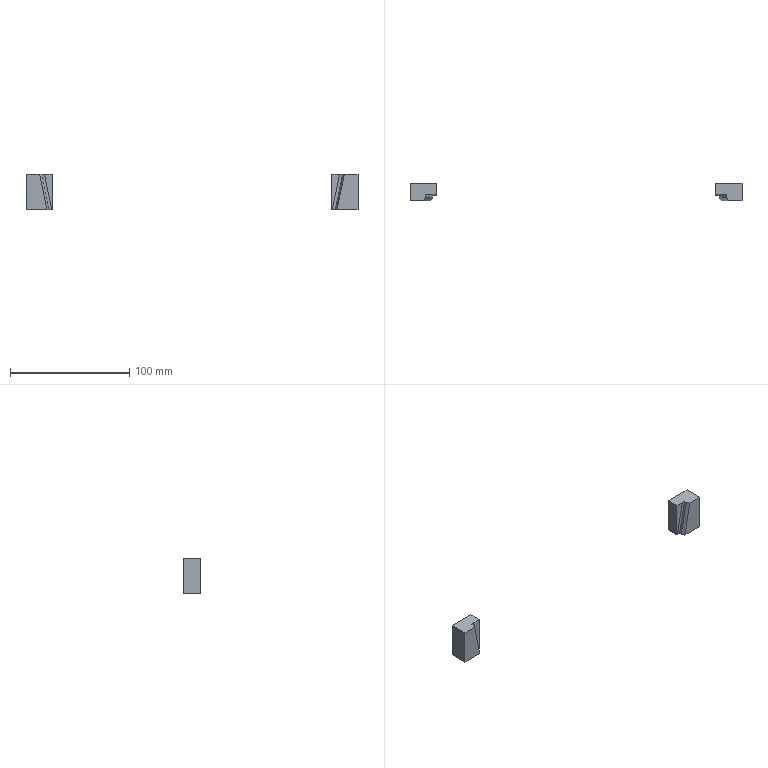Component | SolidWorks | Press-inFixture3-1 | 2 solids | 36 faces | box 278 x 15 x 30 mm | volume 17452 mm3 | plane 20 | cylinder 8 | cone 8 | commonest cylinder face diameters 3.3 x8
STEP:
#1=COLOUR_RGB('',0.7922,0.8196,0.9333);
#2=FILL_AREA_STYLE_COLOUR('',#1);
#3=FILL_AREA_STYLE('',(#2));
#4=SURFACE_STYLE_FILL_AREA(#3);
#5=SURFACE_SIDE_STYLE('',(#4));
#6=SURFACE_STYLE_USAGE(.BOTH.,#5);
#7=PRESENTATION_STYLE_ASSIGNMENT((#6));
#8=CARTESIAN_POINT('',(-3.99,-3.031,7.209));
#9=VERTEX_POINT('',#8);
#10=CARTESIAN_POINT('',(-4.12,-3.031,7.209));
#11=VERTEX_POINT('',#10);
#12=CARTESIAN_POINT('',(-4.055,-3.031,7.209));
#13=DIRECTION('',(-0.,1.,-0.));
#14=DIRECTION('',(-1.,0.,0.));
#15=AXIS2_PLACEMENT_3D('',#12,#13,#14);
#16=CIRCLE('',#15,0.06496);
#17=EDGE_CURVE('',#9,#11,#16,.T.);
#18=ORIENTED_EDGE('',*,*,#17,.F.);
#19=CARTESIAN_POINT('',(-3.99,-2.579,7.209));
#20=VERTEX_POINT('',#19);
#21=CARTESIAN_POINT('',(-3.99,-2.579,7.209));
#22=DIRECTION('',(-0.,1.,-0.));
#23=VECTOR('',#22,39.37);
#24=LINE('',#21,#23);
#25=EDGE_CURVE('',#9,#20,#24,.T.);
#26=ORIENTED_EDGE('',*,*,#25,.T.);
#27=CARTESIAN_POINT('',(-4.12,-2.579,7.209));
#28=VERTEX_POINT('',#27);
#29=CARTESIAN_POINT('',(-4.055,-2.579,7.209));
#30=DIRECTION('',(-0.,1.,-0.));
#31=DIRECTION('',(-1.,0.,0.));
#32=AXIS2_PLACEMENT_3D('',#29,#30,#31);
#33=CIRCLE('',#32,0.06496);
#34=EDGE_CURVE('',#20,#28,#33,.T.);
#35=ORIENTED_EDGE('',*,*,#34,.T.);
#36=CARTESIAN_POINT('',(-4.12,-2.579,7.209));
#37=DIRECTION('',(-0.,1.,-0.));
#38=VECTOR('',#37,39.37);
#39=LINE('',#36,#38);
#40=EDGE_CURVE('',#11,#28,#39,.T.);
#41=ORIENTED_EDGE('',*,*,#40,.F.);
#42=EDGE_LOOP('',(#18,#26,#35,#41));
#43=FACE_OUTER_BOUND('',#42,.T.);
#44=CARTESIAN_POINT('',(-4.055,-2.579,7.209));
#45=DIRECTION('',(-0.,1.,-0.));
#46=DIRECTION('',(-1.,0.,0.));
#47=AXIS2_PLACEMENT_3D('',#44,#45,#46);
#48=CYLINDRICAL_SURFACE('',#47,0.06496);
#49=ADVANCED_FACE('',(#43),#48,.F.);
#50=CARTESIAN_POINT('',(-4.055,-3.071,7.209));
#51=VERTEX_POINT('',#50);
#52=CARTESIAN_POINT('',(-4.12,-3.031,7.209));
#53=DIRECTION('',(-0.8572,0.515,0.));
#54=VECTOR('',#53,39.37);
#55=LINE('',#52,#54);
#56=EDGE_CURVE('',#51,#11,#55,.T.);
#57=ORIENTED_EDGE('',*,*,#56,.F.);
#58=CARTESIAN_POINT('',(-3.99,-3.031,7.209));
#59=DIRECTION('',(0.8572,0.515,-0.));
#60=VECTOR('',#59,39.37);
#61=LINE('',#58,#60);
#62=EDGE_CURVE('',#51,#9,#61,.T.);
#63=ORIENTED_EDGE('',*,*,#62,.T.);
#64=ORIENTED_EDGE('',*,*,#17,.T.);
#65=EDGE_LOOP('',(#57,#63,#64));
#66=FACE_OUTER_BOUND('',#65,.T.);
#67=CARTESIAN_POINT('',(-4.055,-3.031,7.209));
#68=DIRECTION('',(-0.,1.,-0.));
#69=DIRECTION('',(-1.,0.,0.));
#70=AXIS2_PLACEMENT_3D('',#67,#68,#69);
#71=CONICAL_SURFACE('',#70,0.06496,1.03);
#72=ADVANCED_FACE('',(#66),#71,.F.);
#73=CARTESIAN_POINT('',(-3.99,-3.031,6.658));
#74=VERTEX_POINT('',#73);
#75=CARTESIAN_POINT('',(-4.12,-3.031,6.658));
#76=VERTEX_POINT('',#75);
#77=CARTESIAN_POINT('',(-4.055,-3.031,6.658));
#78=DIRECTION('',(-0.,1.,-0.));
#79=DIRECTION('',(-1.,0.,0.));
#80=AXIS2_PLACEMENT_3D('',#77,#78,#79);
#81=CIRCLE('',#80,0.06496);
#82=EDGE_CURVE('',#74,#76,#81,.T.);
#83=ORIENTED_EDGE('',*,*,#82,.F.);
#84=CARTESIAN_POINT('',(-3.99,-2.579,6.658));
#85=VERTEX_POINT('',#84);
#86=CARTESIAN_POINT('',(-3.99,-2.579,6.658));
#87=DIRECTION('',(-0.,1.,-0.));
#88=VECTOR('',#87,39.37);
#89=LINE('',#86,#88);
#90=EDGE_CURVE('',#74,#85,#89,.T.);
#91=ORIENTED_EDGE('',*,*,#90,.T.);
#92=CARTESIAN_POINT('',(-4.12,-2.579,6.658));
#93=VERTEX_POINT('',#92);
#94=CARTESIAN_POINT('',(-4.055,-2.579,6.658));
#95=DIRECTION('',(-0.,1.,-0.));
#96=DIRECTION('',(-1.,0.,0.));
#97=AXIS2_PLACEMENT_3D('',#94,#95,#96);
#98=CIRCLE('',#97,0.06496);
#99=EDGE_CURVE('',#85,#93,#98,.T.);
#100=ORIENTED_EDGE('',*,*,#99,.T.);
#101=CARTESIAN_POINT('',(-4.12,-2.579,6.658));
#102=DIRECTION('',(-0.,1.,-0.));
#103=VECTOR('',#102,39.37);
#104=LINE('',#101,#103);
#105=EDGE_CURVE('',#76,#93,#104,.T.);
#106=ORIENTED_EDGE('',*,*,#105,.F.);
#107=EDGE_LOOP('',(#83,#91,#100,#106));
#108=FACE_OUTER_BOUND('',#107,.T.);
#109=CARTESIAN_POINT('',(-4.055,-2.579,6.658));
#110=DIRECTION('',(-0.,1.,-0.));
#111=DIRECTION('',(-1.,0.,0.));
#112=AXIS2_PLACEMENT_3D('',#109,#110,#111);
#113=CYLINDRICAL_SURFACE('',#112,0.06496);
#114=ADVANCED_FACE('',(#108),#113,.F.);
#115=CARTESIAN_POINT('',(-4.055,-3.071,6.658));
#116=VERTEX_POINT('',#115);
#117=CARTESIAN_POINT('',(-4.12,-3.031,6.658));
#118=DIRECTION('',(-0.8572,0.515,0.));
#119=VECTOR('',#118,39.37);
#120=LINE('',#117,#119);
#121=EDGE_CURVE('',#116,#76,#120,.T.);
#122=ORIENTED_EDGE('',*,*,#121,.F.);
#123=CARTESIAN_POINT('',(-3.99,-3.031,6.658));
#124=DIRECTION('',(0.8572,0.515,-0.));
#125=VECTOR('',#124,39.37);
#126=LINE('',#123,#125);
#127=EDGE_CURVE('',#116,#74,#126,.T.);
#128=ORIENTED_EDGE('',*,*,#127,.T.);
#129=ORIENTED_EDGE('',*,*,#82,.T.);
#130=EDGE_LOOP('',(#122,#128,#129));
#131=FACE_OUTER_BOUND('',#130,.T.);
#132=CARTESIAN_POINT('',(-4.055,-3.031,6.658));
#133=DIRECTION('',(-0.,1.,-0.));
#134=DIRECTION('',(-1.,0.,0.));
#135=AXIS2_PLACEMENT_3D('',#132,#133,#134);
#136=CONICAL_SURFACE('',#135,0.06496,1.03);
#137=ADVANCED_FACE('',(#131),#136,.F.);
#138=CARTESIAN_POINT('',(-3.545,-2.972,6.343));
#139=VERTEX_POINT('',#138);
#140=CARTESIAN_POINT('',(-3.544,-3.051,6.343));
#141=VERTEX_POINT('',#140);
#142=CARTESIAN_POINT('',(-3.542,-3.171,6.343));
#143=DIRECTION('',(0.01741,-0.9998,0.));
#144=VECTOR('',#143,39.37);
#145=LINE('',#142,#144);
#146=EDGE_CURVE('',#139,#141,#145,.T.);
#147=ORIENTED_EDGE('',*,*,#146,.T.);
#148=CARTESIAN_POINT('',(-3.602,-3.169,6.343));
#149=VERTEX_POINT('',#148);
#150=CARTESIAN_POINT('',(-3.6,-3.164,6.343));
#151=DIRECTION('',(-0.4419,-0.8971,0.));
#152=VECTOR('',#151,39.37);
#153=LINE('',#150,#152);
#154=EDGE_CURVE('',#141,#149,#153,.T.);
#155=ORIENTED_EDGE('',*,*,#154,.T.);
#156=CARTESIAN_POINT('',(-4.291,-3.169,6.343));
#157=VERTEX_POINT('',#156);
#158=CARTESIAN_POINT('',(-3.425,-3.169,6.343));
#159=DIRECTION('',(1.,0.,-0.));
#160=VECTOR('',#159,39.37);
#161=LINE('',#158,#160);
#162=EDGE_CURVE('',#157,#149,#161,.T.);
#163=ORIENTED_EDGE('',*,*,#162,.F.);
#164=CARTESIAN_POINT('',(-4.291,-2.579,6.343));
#165=VERTEX_POINT('',#164);
#166=CARTESIAN_POINT('',(-4.291,-3.169,6.343));
#167=DIRECTION('',(-0.,1.,-0.));
#168=VECTOR('',#167,39.37);
#169=LINE('',#166,#168);
#170=EDGE_CURVE('',#157,#165,#169,.T.);
#171=ORIENTED_EDGE('',*,*,#170,.T.);
#172=CARTESIAN_POINT('',(-3.425,-2.579,6.343));
#173=VERTEX_POINT('',#172);
#174=CARTESIAN_POINT('',(-3.425,-2.579,6.343));
#175=DIRECTION('',(1.,0.,-0.));
#176=VECTOR('',#175,39.37);
#177=LINE('',#174,#176);
#178=EDGE_CURVE('',#165,#173,#177,.T.);
#179=ORIENTED_EDGE('',*,*,#178,.T.);
#180=CARTESIAN_POINT('',(-3.425,-2.972,6.343));
#181=VERTEX_POINT('',#180);
#182=CARTESIAN_POINT('',(-3.425,-3.169,6.343));
#183=DIRECTION('',(-0.,1.,-0.));
#184=VECTOR('',#183,39.37);
#185=LINE('',#182,#184);
#186=EDGE_CURVE('',#181,#173,#185,.T.);
#187=ORIENTED_EDGE('',*,*,#186,.F.);
#188=CARTESIAN_POINT('',(-3.445,-2.972,6.343));
#189=VERTEX_POINT('',#188);
#190=CARTESIAN_POINT('',(-3.425,-2.972,6.343));
#191=DIRECTION('',(-1.,0.,0.));
#192=VECTOR('',#191,39.37);
#193=LINE('',#190,#192);
#194=EDGE_CURVE('',#181,#189,#193,.T.);
#195=ORIENTED_EDGE('',*,*,#194,.T.);
#196=CARTESIAN_POINT('',(-3.425,-2.972,6.343));
#197=DIRECTION('',(1.,-0.,-0.));
#198=VECTOR('',#197,39.37);
#199=LINE('',#196,#198);
#200=EDGE_CURVE('',#139,#189,#199,.T.);
#201=ORIENTED_EDGE('',*,*,#200,.F.);
#202=EDGE_LOOP('',(#147,#155,#163,#171,#179,#187,#195,#201));
#203=FACE_OUTER_BOUND('',#202,.T.);
#204=CARTESIAN_POINT('',(-3.425,-3.169,6.343));
#205=DIRECTION('',(0.,0.,1.));
#206=DIRECTION('',(-1.,-0.,0.));
#207=AXIS2_PLACEMENT_3D('',#204,#205,#206);
#208=PLANE('',#207);
#209=ADVANCED_FACE('',(#203),#208,.F.);
#210=CARTESIAN_POINT('',(-3.425,-2.972,7.524));
#211=VERTEX_POINT('',#210);
#212=CARTESIAN_POINT('',(-3.425,-2.579,7.524));
#213=VERTEX_POINT('',#212);
#214=CARTESIAN_POINT('',(-3.425,-3.169,7.524));
#215=DIRECTION('',(-0.,1.,-0.));
#216=VECTOR('',#215,39.37);
#217=LINE('',#214,#216);
#218=EDGE_CURVE('',#211,#213,#217,.T.);
#219=ORIENTED_EDGE('',*,*,#218,.F.);
#220=CARTESIAN_POINT('',(-3.425,-2.972,7.524));
#221=DIRECTION('',(0.,0.,-1.));
#222=VECTOR('',#221,39.37);
#223=LINE('',#220,#222);
#224=EDGE_CURVE('',#211,#181,#223,.T.);
#225=ORIENTED_EDGE('',*,*,#224,.T.);
#226=ORIENTED_EDGE('',*,*,#186,.T.);
#227=CARTESIAN_POINT('',(-3.425,-2.579,7.524));
#228=DIRECTION('',(-0.,0.,1.));
#229=VECTOR('',#228,39.37);
#230=LINE('',#227,#229);
#231=EDGE_CURVE('',#173,#213,#230,.T.);
#232=ORIENTED_EDGE('',*,*,#231,.T.);
#233=EDGE_LOOP('',(#219,#225,#226,#232));
#234=FACE_OUTER_BOUND('',#233,.T.);
#235=CARTESIAN_POINT('',(-3.425,-3.169,7.524));
#236=DIRECTION('',(-1.,-0.,-0.));
#237=DIRECTION('',(0.,-0.,-1.));
#238=AXIS2_PLACEMENT_3D('',#235,#236,#237);
#239=PLANE('',#238);
#240=ADVANCED_FACE('',(#234),#239,.F.);
#241=CARTESIAN_POINT('',(-3.839,-3.169,7.524));
#242=VERTEX_POINT('',#241);
#243=CARTESIAN_POINT('',(-4.291,-3.169,7.524));
#244=VERTEX_POINT('',#243);
#245=CARTESIAN_POINT('',(-3.425,-3.169,7.524));
#246=DIRECTION('',(-1.,-0.,0.));
#247=VECTOR('',#246,39.37);
#248=LINE('',#245,#247);
#249=EDGE_CURVE('',#242,#244,#248,.T.);
#250=ORIENTED_EDGE('',*,*,#249,.F.);
#251=CARTESIAN_POINT('',(-3.781,-3.051,7.524));
#252=VERTEX_POINT('',#251);
#253=CARTESIAN_POINT('',(-3.79,-3.07,7.524));
#254=DIRECTION('',(0.4419,0.8971,-0.));
#255=VECTOR('',#254,39.37);
#256=LINE('',#253,#255);
#257=EDGE_CURVE('',#242,#252,#256,.T.);
#258=ORIENTED_EDGE('',*,*,#257,.T.);
#259=CARTESIAN_POINT('',(-3.782,-2.972,7.524));
#260=VERTEX_POINT('',#259);
#261=CARTESIAN_POINT('',(-3.779,-3.175,7.524));
#262=DIRECTION('',(-0.01741,0.9998,-0.));
#263=VECTOR('',#262,39.37);
#264=LINE('',#261,#263);
#265=EDGE_CURVE('',#252,#260,#264,.T.);
#266=ORIENTED_EDGE('',*,*,#265,.T.);
#267=CARTESIAN_POINT('',(-3.682,-2.972,7.524));
#268=VERTEX_POINT('',#267);
#269=CARTESIAN_POINT('',(-3.425,-2.972,7.524));
#270=DIRECTION('',(-1.,0.,0.));
#271=VECTOR('',#270,39.37);
#272=LINE('',#269,#271);
#273=EDGE_CURVE('',#268,#260,#272,.T.);
#274=ORIENTED_EDGE('',*,*,#273,.F.);
#275=CARTESIAN_POINT('',(-3.425,-2.972,7.524));
#276=DIRECTION('',(1.,-0.,-0.));
#277=VECTOR('',#276,39.37);
#278=LINE('',#275,#277);
#279=EDGE_CURVE('',#268,#211,#278,.T.);
#280=ORIENTED_EDGE('',*,*,#279,.T.);
#281=ORIENTED_EDGE('',*,*,#218,.T.);
#282=CARTESIAN_POINT('',(-4.291,-2.579,7.524));
#283=VERTEX_POINT('',#282);
#284=CARTESIAN_POINT('',(-3.425,-2.579,7.524));
#285=DIRECTION('',(-1.,-0.,0.));
#286=VECTOR('',#285,39.37);
#287=LINE('',#284,#286);
#288=EDGE_CURVE('',#213,#283,#287,.T.);
#289=ORIENTED_EDGE('',*,*,#288,.T.);
#290=CARTESIAN_POINT('',(-4.291,-3.169,7.524));
#291=DIRECTION('',(-0.,1.,-0.));
#292=VECTOR('',#291,39.37);
#293=LINE('',#290,#292);
#294=EDGE_CURVE('',#244,#283,#293,.T.);
#295=ORIENTED_EDGE('',*,*,#294,.F.);
#296=EDGE_LOOP('',(#250,#258,#266,#274,#280,#281,#289,#295));
#297=FACE_OUTER_BOUND('',#296,.T.);
#298=CARTESIAN_POINT('',(-3.425,-3.169,7.524));
#299=DIRECTION('',(-0.,-0.,-1.));
#300=DIRECTION('',(1.,0.,-0.));
#301=AXIS2_PLACEMENT_3D('',#298,#299,#300);
#302=PLANE('',#301);
#303=ADVANCED_FACE('',(#297),#302,.F.);
#304=CARTESIAN_POINT('',(-4.291,-2.579,7.524));
#305=DIRECTION('',(0.,-0.,-1.));
#306=VECTOR('',#305,39.37);
#307=LINE('',#304,#306);
#308=EDGE_CURVE('',#283,#165,#307,.T.);
#309=ORIENTED_EDGE('',*,*,#308,.T.);
#310=ORIENTED_EDGE('',*,*,#170,.F.);
#311=CARTESIAN_POINT('',(-4.291,-3.169,7.524));
#312=DIRECTION('',(0.,-0.,-1.));
#313=VECTOR('',#312,39.37);
#314=LINE('',#311,#313);
#315=EDGE_CURVE('',#244,#157,#314,.T.);
#316=ORIENTED_EDGE('',*,*,#315,.F.);
#317=ORIENTED_EDGE('',*,*,#294,.T.);
#318=EDGE_LOOP('',(#309,#310,#316,#317));
#319=FACE_OUTER_BOUND('',#318,.T.);
#320=CARTESIAN_POINT('',(-4.291,-3.169,7.524));
#321=DIRECTION('',(1.,0.,0.));
#322=DIRECTION('',(-0.,0.,1.));
#323=AXIS2_PLACEMENT_3D('',#320,#321,#322);
#324=PLANE('',#323);
#325=ADVANCED_FACE('',(#319),#324,.F.);
#326=ORIENTED_EDGE('',*,*,#162,.T.);
#327=CARTESIAN_POINT('',(-3.837,-3.169,7.512));
#328=DIRECTION('',(-0.1967,0.,0.9805));
#329=VECTOR('',#328,39.37);
#330=LINE('',#327,#329);
#331=EDGE_CURVE('',#149,#242,#330,.T.);
#332=ORIENTED_EDGE('',*,*,#331,.T.);
#333=ORIENTED_EDGE('',*,*,#249,.T.);
#334=ORIENTED_EDGE('',*,*,#315,.T.);
#335=EDGE_LOOP('',(#326,#332,#333,#334));
#336=FACE_OUTER_BOUND('',#335,.T.);
#337=CARTESIAN_POINT('',(-3.858,-3.169,6.933));
#338=DIRECTION('',(0.,-1.,0.));
#339=DIRECTION('',(1.,0.,-0.));
#340=AXIS2_PLACEMENT_3D('',#337,#338,#339);
#341=PLANE('',#340);
#342=ADVANCED_FACE('',(#336),#341,.T.);
#343=CARTESIAN_POINT('',(-4.055,-2.579,7.209));
#344=DIRECTION('',(-0.,1.,-0.));
#345=DIRECTION('',(-1.,0.,0.));
#346=AXIS2_PLACEMENT_3D('',#343,#344,#345);
#347=CIRCLE('',#346,0.06496);
#348=EDGE_CURVE('',#28,#20,#347,.T.);
#349=ORIENTED_EDGE('',*,*,#348,.F.);
#350=ORIENTED_EDGE('',*,*,#34,.F.);
#351=EDGE_LOOP('',(#349,#350));
#352=FACE_BOUND('',#351,.T.);
#353=CARTESIAN_POINT('',(-4.055,-2.579,6.658));
#354=DIRECTION('',(-0.,1.,-0.));
#355=DIRECTION('',(-1.,0.,0.));
#356=AXIS2_PLACEMENT_3D('',#353,#354,#355);
#357=CIRCLE('',#356,0.06496);
#358=EDGE_CURVE('',#93,#85,#357,.T.);
#359=ORIENTED_EDGE('',*,*,#358,.F.);
#360=ORIENTED_EDGE('',*,*,#99,.F.);
#361=EDGE_LOOP('',(#359,#360));
#362=FACE_BOUND('',#361,.T.);
#363=ORIENTED_EDGE('',*,*,#178,.F.);
#364=ORIENTED_EDGE('',*,*,#308,.F.);
#365=ORIENTED_EDGE('',*,*,#288,.F.);
#366=ORIENTED_EDGE('',*,*,#231,.F.);
#367=EDGE_LOOP('',(#363,#364,#365,#366));
#368=FACE_OUTER_BOUND('',#367,.T.);
#369=CARTESIAN_POINT('',(-3.858,-2.579,6.933));
#370=DIRECTION('',(0.,-1.,0.));
#371=DIRECTION('',(1.,0.,-0.));
#372=AXIS2_PLACEMENT_3D('',#369,#370,#371);
#373=PLANE('',#372);
#374=ADVANCED_FACE('',(#352,#362,#368),#373,.F.);
#375=ORIENTED_EDGE('',*,*,#194,.F.);
#376=ORIENTED_EDGE('',*,*,#224,.F.);
#377=ORIENTED_EDGE('',*,*,#279,.F.);
#378=CARTESIAN_POINT('',(-3.747,-2.972,7.85));
#379=DIRECTION('',(-0.1967,0.,0.9805));
#380=VECTOR('',#379,39.37);
#381=LINE('',#378,#380);
#382=EDGE_CURVE('',#189,#268,#381,.T.);
#383=ORIENTED_EDGE('',*,*,#382,.F.);
#384=EDGE_LOOP('',(#375,#376,#377,#383));
#385=FACE_OUTER_BOUND('',#384,.T.);
#386=CARTESIAN_POINT('',(-3.355,-2.972,6.018));
#387=DIRECTION('',(0.,1.,0.));
#388=DIRECTION('',(1.,-0.,0.));
#389=AXIS2_PLACEMENT_3D('',#386,#387,#388);
#390=PLANE('',#389);
#391=ADVANCED_FACE('',(#385),#390,.F.);
#392=CARTESIAN_POINT('',(-3.83,-2.972,7.763));
#393=DIRECTION('',(0.1967,-0.,-0.9805));
#394=VECTOR('',#393,39.37);
#395=LINE('',#392,#394);
#396=EDGE_CURVE('',#260,#139,#395,.T.);
#397=ORIENTED_EDGE('',*,*,#396,.T.);
#398=ORIENTED_EDGE('',*,*,#200,.T.);
#399=ORIENTED_EDGE('',*,*,#382,.T.);
#400=ORIENTED_EDGE('',*,*,#273,.T.);
#401=EDGE_LOOP('',(#397,#398,#399,#400));
#402=FACE_OUTER_BOUND('',#401,.T.);
#403=CARTESIAN_POINT('',(-1.579,-2.972,7.058));
#404=DIRECTION('',(-0.,-1.,0.));
#405=DIRECTION('',(-0.,0.,1.));
#406=AXIS2_PLACEMENT_3D('',#403,#404,#405);
#407=PLANE('',#406);
#408=ADVANCED_FACE('',(#402),#407,.T.);
#409=ORIENTED_EDGE('',*,*,#265,.F.);
#410=CARTESIAN_POINT('',(-3.544,-3.051,6.342));
#411=DIRECTION('',(0.1967,-0.,-0.9805));
#412=VECTOR('',#411,39.37);
#413=LINE('',#410,#412);
#414=EDGE_CURVE('',#252,#141,#413,.T.);
#415=ORIENTED_EDGE('',*,*,#414,.T.);
#416=ORIENTED_EDGE('',*,*,#146,.F.);
#417=ORIENTED_EDGE('',*,*,#396,.F.);
#418=EDGE_LOOP('',(#409,#415,#416,#417));
#419=FACE_OUTER_BOUND('',#418,.T.);
#420=CARTESIAN_POINT('',(-3.798,-4.876,7.765));
#421=DIRECTION('',(-0.9803,-0.01707,-0.1966));
#422=DIRECTION('',(-0.01745,0.9998,0.000201));
#423=AXIS2_PLACEMENT_3D('',#420,#421,#422);
#424=PLANE('',#423);
#425=ADVANCED_FACE('',(#419),#424,.F.);
#426=ORIENTED_EDGE('',*,*,#127,.F.);
#427=ORIENTED_EDGE('',*,*,#121,.T.);
#428=CARTESIAN_POINT('',(-4.055,-3.031,6.658));
#429=DIRECTION('',(-0.,1.,-0.));
#430=DIRECTION('',(-1.,0.,0.));
#431=AXIS2_PLACEMENT_3D('',#428,#429,#430);
#432=CIRCLE('',#431,0.06496);
#433=EDGE_CURVE('',#76,#74,#432,.T.);
#434=ORIENTED_EDGE('',*,*,#433,.T.);
#435=EDGE_LOOP('',(#426,#427,#434));
#436=FACE_OUTER_BOUND('',#435,.T.);
#437=CARTESIAN_POINT('',(-4.055,-3.031,6.658));
#438=DIRECTION('',(-0.,1.,-0.));
#439=DIRECTION('',(-1.,0.,0.));
#440=AXIS2_PLACEMENT_3D('',#437,#438,#439);
#441=CONICAL_SURFACE('',#440,0.06496,1.03);
#442=ADVANCED_FACE('',(#436),#441,.F.);
#443=ORIENTED_EDGE('',*,*,#90,.F.);
#444=ORIENTED_EDGE('',*,*,#433,.F.);
#445=ORIENTED_EDGE('',*,*,#105,.T.);
#446=ORIENTED_EDGE('',*,*,#358,.T.);
#447=EDGE_LOOP('',(#443,#444,#445,#446));
#448=FACE_OUTER_BOUND('',#447,.T.);
#449=CARTESIAN_POINT('',(-4.055,-2.579,6.658));
#450=DIRECTION('',(-0.,1.,-0.));
#451=DIRECTION('',(-1.,0.,0.));
#452=AXIS2_PLACEMENT_3D('',#449,#450,#451);
#453=CYLINDRICAL_SURFACE('',#452,0.06496);
#454=ADVANCED_FACE('',(#448),#453,.F.);
#455=ORIENTED_EDGE('',*,*,#62,.F.);
#456=ORIENTED_EDGE('',*,*,#56,.T.);
#457=CARTESIAN_POINT('',(-4.055,-3.031,7.209));
#458=DIRECTION('',(-0.,1.,-0.));
#459=DIRECTION('',(-1.,0.,0.));
#460=AXIS2_PLACEMENT_3D('',#457,#458,#459);
#461=CIRCLE('',#460,0.06496);
#462=EDGE_CURVE('',#11,#9,#461,.T.);
#463=ORIENTED_EDGE('',*,*,#462,.T.);
#464=EDGE_LOOP('',(#455,#456,#463));
#465=FACE_OUTER_BOUND('',#464,.T.);
#466=CARTESIAN_POINT('',(-4.055,-3.031,7.209));
#467=DIRECTION('',(-0.,1.,-0.));
#468=DIRECTION('',(-1.,0.,0.));
#469=AXIS2_PLACEMENT_3D('',#466,#467,#468);
#470=CONICAL_SURFACE('',#469,0.06496,1.03);
#471=ADVANCED_FACE('',(#465),#470,.F.);
#472=ORIENTED_EDGE('',*,*,#25,.F.);
#473=ORIENTED_EDGE('',*,*,#462,.F.);
#474=ORIENTED_EDGE('',*,*,#40,.T.);
#475=ORIENTED_EDGE('',*,*,#348,.T.);
#476=EDGE_LOOP('',(#472,#473,#474,#475));
#477=FACE_OUTER_BOUND('',#476,.T.);
#478=CARTESIAN_POINT('',(-4.055,-2.579,7.209));
#479=DIRECTION('',(-0.,1.,-0.));
#480=DIRECTION('',(-1.,0.,0.));
#481=AXIS2_PLACEMENT_3D('',#478,#479,#480);
#482=CYLINDRICAL_SURFACE('',#481,0.06496);
#483=ADVANCED_FACE('',(#477),#482,.F.);
#484=ORIENTED_EDGE('',*,*,#257,.F.);
#485=ORIENTED_EDGE('',*,*,#331,.F.);
#486=ORIENTED_EDGE('',*,*,#154,.F.);
#487=ORIENTED_EDGE('',*,*,#414,.F.);
#488=EDGE_LOOP('',(#484,#485,#486,#487));
#489=FACE_OUTER_BOUND('',#488,.T.);
#490=CARTESIAN_POINT('',(-3.828,-3.051,7.759));
#491=DIRECTION('',(0.8829,-0.4349,0.1771));
#492=DIRECTION('',(-0.1967,0.,0.9805));
#493=AXIS2_PLACEMENT_3D('',#490,#491,#492);
#494=PLANE('',#493);
#495=ADVANCED_FACE('',(#489),#494,.T.);
#496=CLOSED_SHELL('',(#49,#72,#114,#137,#209,#240,#303,#325,#342,#374,#391,#408,#425,#442,#454,#471,#483,#495));
#497=MANIFOLD_SOLID_BREP('',#496);
#498=STYLED_ITEM('',(#7),#497);
#499=(LENGTH_UNIT()NAMED_UNIT(*)SI_UNIT($,.METRE.));
#500=LENGTH_MEASURE_WITH_UNIT(LENGTH_MEASURE(0.0254),#499);
#501=DIMENSIONAL_EXPONENTS(1.,0.,0.,0.,0.,0.,0.);
#502=(CONVERSION_BASED_UNIT('',#500)LENGTH_UNIT()NAMED_UNIT(#501));
#503=UNCERTAINTY_MEASURE_WITH_UNIT(LENGTH_MEASURE(0.00001),#502,'','');
#504=(NAMED_UNIT(*)PLANE_ANGLE_UNIT()SI_UNIT($,.RADIAN.));
#505=(NAMED_UNIT(*)SI_UNIT($,.STERADIAN.)SOLID_ANGLE_UNIT());
#506=(GEOMETRIC_REPRESENTATION_CONTEXT(3)GLOBAL_UNCERTAINTY_ASSIGNED_CONTEXT((#503))GLOBAL_UNIT_ASSIGNED_CONTEXT((#502,#504,#505))REPRESENTATION_CONTEXT('',''));
#507=MECHANICAL_DESIGN_GEOMETRIC_PRESENTATION_REPRESENTATION('',(#498),#506);
#508=CARTESIAN_POINT('',(6.482,-3.031,7.209));
#509=VERTEX_POINT('',#508);
#510=CARTESIAN_POINT('',(6.352,-3.031,7.209));
#511=VERTEX_POINT('',#510);
#512=CARTESIAN_POINT('',(6.417,-3.031,7.209));
#513=DIRECTION('',(-0.,-1.,0.));
#514=DIRECTION('',(1.,0.,0.));
#515=AXIS2_PLACEMENT_3D('',#512,#513,#514);
#516=CIRCLE('',#515,0.06496);
#517=EDGE_CURVE('',#509,#511,#516,.T.);
#518=ORIENTED_EDGE('',*,*,#517,.T.);
#519=CARTESIAN_POINT('',(6.352,-2.579,7.209));
#520=VERTEX_POINT('',#519);
#521=CARTESIAN_POINT('',(6.352,-2.579,7.209));
#522=DIRECTION('',(0.,1.,-0.));
#523=VECTOR('',#522,39.37);
#524=LINE('',#521,#523);
#525=EDGE_CURVE('',#511,#520,#524,.T.);
#526=ORIENTED_EDGE('',*,*,#525,.T.);
#527=CARTESIAN_POINT('',(6.482,-2.579,7.209));
#528=VERTEX_POINT('',#527);
#529=CARTESIAN_POINT('',(6.417,-2.579,7.209));
#530=DIRECTION('',(-0.,-1.,0.));
#531=DIRECTION('',(1.,0.,0.));
#532=AXIS2_PLACEMENT_3D('',#529,#530,#531);
#533=CIRCLE('',#532,0.06496);
#534=EDGE_CURVE('',#528,#520,#533,.T.);
#535=ORIENTED_EDGE('',*,*,#534,.F.);
#536=CARTESIAN_POINT('',(6.482,-2.579,7.209));
#537=DIRECTION('',(0.,1.,-0.));
#538=VECTOR('',#537,39.37);
#539=LINE('',#536,#538);
#540=EDGE_CURVE('',#509,#528,#539,.T.);
#541=ORIENTED_EDGE('',*,*,#540,.F.);
#542=EDGE_LOOP('',(#518,#526,#535,#541));
#543=FACE_OUTER_BOUND('',#542,.T.);
#544=CARTESIAN_POINT('',(6.417,-2.579,7.209));
#545=DIRECTION('',(0.,1.,-0.));
#546=DIRECTION('',(1.,0.,0.));
#547=AXIS2_PLACEMENT_3D('',#544,#545,#546);
#548=CYLINDRICAL_SURFACE('',#547,0.06496);
#549=ADVANCED_FACE('',(#543),#548,.F.);
#550=CARTESIAN_POINT('',(6.417,-3.071,7.209));
#551=VERTEX_POINT('',#550);
#552=CARTESIAN_POINT('',(6.482,-3.031,7.209));
#553=DIRECTION('',(0.8572,0.515,0.));
#554=VECTOR('',#553,39.37);
#555=LINE('',#552,#554);
#556=EDGE_CURVE('',#551,#509,#555,.T.);
#557=ORIENTED_EDGE('',*,*,#556,.F.);
#558=CARTESIAN_POINT('',(6.352,-3.031,7.209));
#559=DIRECTION('',(-0.8572,0.515,-0.));
#560=VECTOR('',#559,39.37);
#561=LINE('',#558,#560);
#562=EDGE_CURVE('',#551,#511,#561,.T.);
#563=ORIENTED_EDGE('',*,*,#562,.T.);
#564=ORIENTED_EDGE('',*,*,#517,.F.);
#565=EDGE_LOOP('',(#557,#563,#564));
#566=FACE_OUTER_BOUND('',#565,.T.);
#567=CARTESIAN_POINT('',(6.417,-3.031,7.209));
#568=DIRECTION('',(0.,1.,-0.));
#569=DIRECTION('',(1.,0.,0.));
#570=AXIS2_PLACEMENT_3D('',#567,#568,#569);
#571=CONICAL_SURFACE('',#570,0.06496,1.03);
#572=ADVANCED_FACE('',(#566),#571,.F.);
#573=CARTESIAN_POINT('',(6.482,-3.031,6.658));
#574=VERTEX_POINT('',#573);
#575=CARTESIAN_POINT('',(6.352,-3.031,6.658));
#576=VERTEX_POINT('',#575);
#577=CARTESIAN_POINT('',(6.417,-3.031,6.658));
#578=DIRECTION('',(-0.,-1.,0.));
#579=DIRECTION('',(1.,0.,0.));
#580=AXIS2_PLACEMENT_3D('',#577,#578,#579);
#581=CIRCLE('',#580,0.06496);
#582=EDGE_CURVE('',#574,#576,#581,.T.);
#583=ORIENTED_EDGE('',*,*,#582,.T.);
#584=CARTESIAN_POINT('',(6.352,-2.579,6.658));
#585=VERTEX_POINT('',#584);
#586=CARTESIAN_POINT('',(6.352,-2.579,6.658));
#587=DIRECTION('',(0.,1.,-0.));
#588=VECTOR('',#587,39.37);
#589=LINE('',#586,#588);
#590=EDGE_CURVE('',#576,#585,#589,.T.);
#591=ORIENTED_EDGE('',*,*,#590,.T.);
#592=CARTESIAN_POINT('',(6.482,-2.579,6.658));
#593=VERTEX_POINT('',#592);
#594=CARTESIAN_POINT('',(6.417,-2.579,6.658));
#595=DIRECTION('',(-0.,-1.,0.));
#596=DIRECTION('',(1.,0.,0.));
#597=AXIS2_PLACEMENT_3D('',#594,#595,#596);
#598=CIRCLE('',#597,0.06496);
#599=EDGE_CURVE('',#593,#585,#598,.T.);
#600=ORIENTED_EDGE('',*,*,#599,.F.);
#601=CARTESIAN_POINT('',(6.482,-2.579,6.658));
#602=DIRECTION('',(0.,1.,-0.));
#603=VECTOR('',#602,39.37);
#604=LINE('',#601,#603);
#605=EDGE_CURVE('',#574,#593,#604,.T.);
#606=ORIENTED_EDGE('',*,*,#605,.F.);
#607=EDGE_LOOP('',(#583,#591,#600,#606));
#608=FACE_OUTER_BOUND('',#607,.T.);
#609=CARTESIAN_POINT('',(6.417,-2.579,6.658));
#610=DIRECTION('',(0.,1.,-0.));
#611=DIRECTION('',(1.,0.,0.));
#612=AXIS2_PLACEMENT_3D('',#609,#610,#611);
#613=CYLINDRICAL_SURFACE('',#612,0.06496);
#614=ADVANCED_FACE('',(#608),#613,.F.);
#615=CARTESIAN_POINT('',(6.417,-3.071,6.658));
#616=VERTEX_POINT('',#615);
#617=CARTESIAN_POINT('',(6.482,-3.031,6.658));
#618=DIRECTION('',(0.8572,0.515,0.));
#619=VECTOR('',#618,39.37);
#620=LINE('',#617,#619);
#621=EDGE_CURVE('',#616,#574,#620,.T.);
#622=ORIENTED_EDGE('',*,*,#621,.F.);
#623=CARTESIAN_POINT('',(6.352,-3.031,6.658));
#624=DIRECTION('',(-0.8572,0.515,-0.));
#625=VECTOR('',#624,39.37);
#626=LINE('',#623,#625);
#627=EDGE_CURVE('',#616,#576,#626,.T.);
#628=ORIENTED_EDGE('',*,*,#627,.T.);
#629=ORIENTED_EDGE('',*,*,#582,.F.);
#630=EDGE_LOOP('',(#622,#628,#629));
#631=FACE_OUTER_BOUND('',#630,.T.);
#632=CARTESIAN_POINT('',(6.417,-3.031,6.658));
#633=DIRECTION('',(0.,1.,-0.));
#634=DIRECTION('',(1.,0.,0.));
#635=AXIS2_PLACEMENT_3D('',#632,#633,#634);
#636=CONICAL_SURFACE('',#635,0.06496,1.03);
#637=ADVANCED_FACE('',(#631),#636,.F.);
#638=CARTESIAN_POINT('',(5.908,-2.972,6.343));
#639=VERTEX_POINT('',#638);
#640=CARTESIAN_POINT('',(5.906,-3.051,6.343));
#641=VERTEX_POINT('',#640);
#642=CARTESIAN_POINT('',(5.904,-3.171,6.343));
#643=DIRECTION('',(-0.01741,-0.9998,0.));
#644=VECTOR('',#643,39.37);
#645=LINE('',#642,#644);
#646=EDGE_CURVE('',#639,#641,#645,.T.);
#647=ORIENTED_EDGE('',*,*,#646,.F.);
#648=CARTESIAN_POINT('',(5.807,-2.972,6.343));
#649=VERTEX_POINT('',#648);
#650=CARTESIAN_POINT('',(5.787,-2.972,6.343));
#651=DIRECTION('',(-1.,0.,-0.));
#652=VECTOR('',#651,39.37);
#653=LINE('',#650,#652);
#654=EDGE_CURVE('',#639,#649,#653,.T.);
#655=ORIENTED_EDGE('',*,*,#654,.T.);
#656=CARTESIAN_POINT('',(5.787,-2.972,6.343));
#657=VERTEX_POINT('',#656);
#658=CARTESIAN_POINT('',(5.787,-2.972,6.343));
#659=DIRECTION('',(1.,0.,0.));
#660=VECTOR('',#659,39.37);
#661=LINE('',#658,#660);
#662=EDGE_CURVE('',#657,#649,#661,.T.);
#663=ORIENTED_EDGE('',*,*,#662,.F.);
#664=CARTESIAN_POINT('',(5.787,-2.579,6.343));
#665=VERTEX_POINT('',#664);
#666=CARTESIAN_POINT('',(5.787,-3.169,6.343));
#667=DIRECTION('',(0.,1.,-0.));
#668=VECTOR('',#667,39.37);
#669=LINE('',#666,#668);
#670=EDGE_CURVE('',#657,#665,#669,.T.);
#671=ORIENTED_EDGE('',*,*,#670,.T.);
#672=CARTESIAN_POINT('',(6.654,-2.579,6.343));
#673=VERTEX_POINT('',#672);
#674=CARTESIAN_POINT('',(5.787,-2.579,6.343));
#675=DIRECTION('',(-1.,0.,-0.));
#676=VECTOR('',#675,39.37);
#677=LINE('',#674,#676);
#678=EDGE_CURVE('',#673,#665,#677,.T.);
#679=ORIENTED_EDGE('',*,*,#678,.F.);
#680=CARTESIAN_POINT('',(6.654,-3.169,6.343));
#681=VERTEX_POINT('',#680);
#682=CARTESIAN_POINT('',(6.654,-3.169,6.343));
#683=DIRECTION('',(0.,1.,-0.));
#684=VECTOR('',#683,39.37);
#685=LINE('',#682,#684);
#686=EDGE_CURVE('',#681,#673,#685,.T.);
#687=ORIENTED_EDGE('',*,*,#686,.F.);
#688=CARTESIAN_POINT('',(5.964,-3.169,6.343));
#689=VERTEX_POINT('',#688);
#690=CARTESIAN_POINT('',(5.787,-3.169,6.343));
#691=DIRECTION('',(-1.,0.,-0.));
#692=VECTOR('',#691,39.37);
#693=LINE('',#690,#692);
#694=EDGE_CURVE('',#681,#689,#693,.T.);
#695=ORIENTED_EDGE('',*,*,#694,.T.);
#696=CARTESIAN_POINT('',(5.962,-3.164,6.343));
#697=DIRECTION('',(0.4419,-0.8971,0.));
#698=VECTOR('',#697,39.37);
#699=LINE('',#696,#698);
#700=EDGE_CURVE('',#641,#689,#699,.T.);
#701=ORIENTED_EDGE('',*,*,#700,.F.);
#702=EDGE_LOOP('',(#647,#655,#663,#671,#679,#687,#695,#701));
#703=FACE_OUTER_BOUND('',#702,.T.);
#704=CARTESIAN_POINT('',(5.787,-3.169,6.343));
#705=DIRECTION('',(-0.,0.,1.));
#706=DIRECTION('',(1.,-0.,0.));
#707=AXIS2_PLACEMENT_3D('',#704,#705,#706);
#708=PLANE('',#707);
#709=ADVANCED_FACE('',(#703),#708,.F.);
#710=CARTESIAN_POINT('',(5.787,-2.972,7.524));
#711=VERTEX_POINT('',#710);
#712=CARTESIAN_POINT('',(5.787,-2.579,7.524));
#713=VERTEX_POINT('',#712);
#714=CARTESIAN_POINT('',(5.787,-3.169,7.524));
#715=DIRECTION('',(0.,1.,-0.));
#716=VECTOR('',#715,39.37);
#717=LINE('',#714,#716);
#718=EDGE_CURVE('',#711,#713,#717,.T.);
#719=ORIENTED_EDGE('',*,*,#718,.T.);
#720=CARTESIAN_POINT('',(5.787,-2.579,7.524));
#721=DIRECTION('',(-0.,0.,1.));
#722=VECTOR('',#721,39.37);
#723=LINE('',#720,#722);
#724=EDGE_CURVE('',#665,#713,#723,.T.);
#725=ORIENTED_EDGE('',*,*,#724,.F.);
#726=ORIENTED_EDGE('',*,*,#670,.F.);
#727=CARTESIAN_POINT('',(5.787,-2.972,7.524));
#728=DIRECTION('',(0.,0.,-1.));
#729=VECTOR('',#728,39.37);
#730=LINE('',#727,#729);
#731=EDGE_CURVE('',#711,#657,#730,.T.);
#732=ORIENTED_EDGE('',*,*,#731,.F.);
#733=EDGE_LOOP('',(#719,#725,#726,#732));
#734=FACE_OUTER_BOUND('',#733,.T.);
#735=CARTESIAN_POINT('',(5.787,-3.169,7.524));
#736=DIRECTION('',(1.,-0.,0.));
#737=DIRECTION('',(0.,-0.,-1.));
#738=AXIS2_PLACEMENT_3D('',#735,#736,#737);
#739=PLANE('',#738);
#740=ADVANCED_FACE('',(#734),#739,.F.);
#741=CARTESIAN_POINT('',(6.201,-3.169,7.524));
#742=VERTEX_POINT('',#741);
#743=CARTESIAN_POINT('',(6.654,-3.169,7.524));
#744=VERTEX_POINT('',#743);
#745=CARTESIAN_POINT('',(5.787,-3.169,7.524));
#746=DIRECTION('',(1.,-0.,0.));
#747=VECTOR('',#746,39.37);
#748=LINE('',#745,#747);
#749=EDGE_CURVE('',#742,#744,#748,.T.);
#750=ORIENTED_EDGE('',*,*,#749,.T.);
#751=CARTESIAN_POINT('',(6.654,-2.579,7.524));
#752=VERTEX_POINT('',#751);
#753=CARTESIAN_POINT('',(6.654,-3.169,7.524));
#754=DIRECTION('',(0.,1.,-0.));
#755=VECTOR('',#754,39.37);
#756=LINE('',#753,#755);
#757=EDGE_CURVE('',#744,#752,#756,.T.);
#758=ORIENTED_EDGE('',*,*,#757,.T.);
#759=CARTESIAN_POINT('',(5.787,-2.579,7.524));
#760=DIRECTION('',(1.,-0.,0.));
#761=VECTOR('',#760,39.37);
#762=LINE('',#759,#761);
#763=EDGE_CURVE('',#713,#752,#762,.T.);
#764=ORIENTED_EDGE('',*,*,#763,.F.);
#765=ORIENTED_EDGE('',*,*,#718,.F.);
#766=CARTESIAN_POINT('',(6.044,-2.972,7.524));
#767=VERTEX_POINT('',#766);
#768=CARTESIAN_POINT('',(5.787,-2.972,7.524));
#769=DIRECTION('',(-1.,-0.,-0.));
#770=VECTOR('',#769,39.37);
#771=LINE('',#768,#770);
#772=EDGE_CURVE('',#767,#711,#771,.T.);
#773=ORIENTED_EDGE('',*,*,#772,.F.);
#774=CARTESIAN_POINT('',(6.145,-2.972,7.524));
#775=VERTEX_POINT('',#774);
#776=CARTESIAN_POINT('',(5.787,-2.972,7.524));
#777=DIRECTION('',(1.,-0.,0.));
#778=VECTOR('',#777,39.37);
#779=LINE('',#776,#778);
#780=EDGE_CURVE('',#767,#775,#779,.T.);
#781=ORIENTED_EDGE('',*,*,#780,.T.);
#782=CARTESIAN_POINT('',(6.143,-3.051,7.524));
#783=VERTEX_POINT('',#782);
#784=CARTESIAN_POINT('',(6.141,-3.175,7.524));
#785=DIRECTION('',(0.01741,0.9998,-0.));
#786=VECTOR('',#785,39.37);
#787=LINE('',#784,#786);
#788=EDGE_CURVE('',#783,#775,#787,.T.);
#789=ORIENTED_EDGE('',*,*,#788,.F.);
#790=CARTESIAN_POINT('',(6.152,-3.07,7.524));
#791=DIRECTION('',(-0.4419,0.8971,-0.));
#792=VECTOR('',#791,39.37);
#793=LINE('',#790,#792);
#794=EDGE_CURVE('',#742,#783,#793,.T.);
#795=ORIENTED_EDGE('',*,*,#794,.F.);
#796=EDGE_LOOP('',(#750,#758,#764,#765,#773,#781,#789,#795));
#797=FACE_OUTER_BOUND('',#796,.T.);
#798=CARTESIAN_POINT('',(5.787,-3.169,7.524));
#799=DIRECTION('',(0.,-0.,-1.));
#800=DIRECTION('',(-1.,0.,-0.));
#801=AXIS2_PLACEMENT_3D('',#798,#799,#800);
#802=PLANE('',#801);
#803=ADVANCED_FACE('',(#797),#802,.F.);
#804=CARTESIAN_POINT('',(6.654,-2.579,7.524));
#805=DIRECTION('',(0.,-0.,-1.));
#806=VECTOR('',#805,39.37);
#807=LINE('',#804,#806);
#808=EDGE_CURVE('',#752,#673,#807,.T.);
#809=ORIENTED_EDGE('',*,*,#808,.F.);
#810=ORIENTED_EDGE('',*,*,#757,.F.);
#811=CARTESIAN_POINT('',(6.654,-3.169,7.524));
#812=DIRECTION('',(0.,-0.,-1.));
#813=VECTOR('',#812,39.37);
#814=LINE('',#811,#813);
#815=EDGE_CURVE('',#744,#681,#814,.T.);
#816=ORIENTED_EDGE('',*,*,#815,.T.);
#817=ORIENTED_EDGE('',*,*,#686,.T.);
#818=EDGE_LOOP('',(#809,#810,#816,#817));
#819=FACE_OUTER_BOUND('',#818,.T.);
#820=CARTESIAN_POINT('',(6.654,-3.169,7.524));
#821=DIRECTION('',(-1.,0.,-0.));
#822=DIRECTION('',(-0.,0.,1.));
#823=AXIS2_PLACEMENT_3D('',#820,#821,#822);
#824=PLANE('',#823);
#825=ADVANCED_FACE('',(#819),#824,.F.);
#826=ORIENTED_EDGE('',*,*,#694,.F.);
#827=ORIENTED_EDGE('',*,*,#815,.F.);
#828=ORIENTED_EDGE('',*,*,#749,.F.);
#829=CARTESIAN_POINT('',(6.199,-3.169,7.512));
#830=DIRECTION('',(0.1967,0.,0.9805));
#831=VECTOR('',#830,39.37);
#832=LINE('',#829,#831);
#833=EDGE_CURVE('',#689,#742,#832,.T.);
#834=ORIENTED_EDGE('',*,*,#833,.F.);
#835=EDGE_LOOP('',(#826,#827,#828,#834));
#836=FACE_OUTER_BOUND('',#835,.T.);
#837=CARTESIAN_POINT('',(6.22,-3.169,6.933));
#838=DIRECTION('',(-0.,-1.,0.));
#839=DIRECTION('',(-1.,0.,-0.));
#840=AXIS2_PLACEMENT_3D('',#837,#838,#839);
#841=PLANE('',#840);
#842=ADVANCED_FACE('',(#836),#841,.T.);
#843=ORIENTED_EDGE('',*,*,#534,.T.);
#844=CARTESIAN_POINT('',(6.417,-2.579,7.209));
#845=DIRECTION('',(-0.,-1.,0.));
#846=DIRECTION('',(1.,0.,0.));
#847=AXIS2_PLACEMENT_3D('',#844,#845,#846);
#848=CIRCLE('',#847,0.06496);
#849=EDGE_CURVE('',#520,#528,#848,.T.);
#850=ORIENTED_EDGE('',*,*,#849,.T.);
#851=EDGE_LOOP('',(#843,#850));
#852=FACE_BOUND('',#851,.T.);
#853=ORIENTED_EDGE('',*,*,#599,.T.);
#854=CARTESIAN_POINT('',(6.417,-2.579,6.658));
#855=DIRECTION('',(-0.,-1.,0.));
#856=DIRECTION('',(1.,0.,0.));
#857=AXIS2_PLACEMENT_3D('',#854,#855,#856);
#858=CIRCLE('',#857,0.06496);
#859=EDGE_CURVE('',#585,#593,#858,.T.);
#860=ORIENTED_EDGE('',*,*,#859,.T.);
#861=EDGE_LOOP('',(#853,#860));
#862=FACE_BOUND('',#861,.T.);
#863=ORIENTED_EDGE('',*,*,#678,.T.);
#864=ORIENTED_EDGE('',*,*,#724,.T.);
#865=ORIENTED_EDGE('',*,*,#763,.T.);
#866=ORIENTED_EDGE('',*,*,#808,.T.);
#867=EDGE_LOOP('',(#863,#864,#865,#866));
#868=FACE_OUTER_BOUND('',#867,.T.);
#869=CARTESIAN_POINT('',(6.22,-2.579,6.933));
#870=DIRECTION('',(-0.,-1.,0.));
#871=DIRECTION('',(-1.,0.,-0.));
#872=AXIS2_PLACEMENT_3D('',#869,#870,#871);
#873=PLANE('',#872);
#874=ADVANCED_FACE('',(#852,#862,#868),#873,.F.);
#875=ORIENTED_EDGE('',*,*,#662,.T.);
#876=CARTESIAN_POINT('',(6.11,-2.972,7.85));
#877=DIRECTION('',(0.1967,0.,0.9805));
#878=VECTOR('',#877,39.37);
#879=LINE('',#876,#878);
#880=EDGE_CURVE('',#649,#767,#879,.T.);
#881=ORIENTED_EDGE('',*,*,#880,.T.);
#882=ORIENTED_EDGE('',*,*,#772,.T.);
#883=ORIENTED_EDGE('',*,*,#731,.T.);
#884=EDGE_LOOP('',(#875,#881,#882,#883));
#885=FACE_OUTER_BOUND('',#884,.T.);
#886=CARTESIAN_POINT('',(5.717,-2.972,6.018));
#887=DIRECTION('',(-0.,1.,0.));
#888=DIRECTION('',(-1.,-0.,0.));
#889=AXIS2_PLACEMENT_3D('',#886,#887,#888);
#890=PLANE('',#889);
#891=ADVANCED_FACE('',(#885),#890,.F.);
#892=CARTESIAN_POINT('',(6.193,-2.972,7.763));
#893=DIRECTION('',(-0.1967,-0.,-0.9805));
#894=VECTOR('',#893,39.37);
#895=LINE('',#892,#894);
#896=EDGE_CURVE('',#775,#639,#895,.T.);
#897=ORIENTED_EDGE('',*,*,#896,.F.);
#898=ORIENTED_EDGE('',*,*,#780,.F.);
#899=ORIENTED_EDGE('',*,*,#880,.F.);
#900=ORIENTED_EDGE('',*,*,#654,.F.);
#901=EDGE_LOOP('',(#897,#898,#899,#900));
#902=FACE_OUTER_BOUND('',#901,.T.);
#903=CARTESIAN_POINT('',(3.941,-2.972,7.058));
#904=DIRECTION('',(-0.,-1.,0.));
#905=DIRECTION('',(-0.,0.,1.));
#906=AXIS2_PLACEMENT_3D('',#903,#904,#905);
#907=PLANE('',#906);
#908=ADVANCED_FACE('',(#902),#907,.T.);
#909=ORIENTED_EDGE('',*,*,#788,.T.);
#910=ORIENTED_EDGE('',*,*,#896,.T.);
#911=ORIENTED_EDGE('',*,*,#646,.T.);
#912=CARTESIAN_POINT('',(5.906,-3.051,6.342));
#913=DIRECTION('',(-0.1967,-0.,-0.9805));
#914=VECTOR('',#913,39.37);
#915=LINE('',#912,#914);
#916=EDGE_CURVE('',#783,#641,#915,.T.);
#917=ORIENTED_EDGE('',*,*,#916,.F.);
#918=EDGE_LOOP('',(#909,#910,#911,#917));
#919=FACE_OUTER_BOUND('',#918,.T.);
#920=CARTESIAN_POINT('',(6.16,-4.876,7.765));
#921=DIRECTION('',(0.9803,-0.01707,-0.1966));
#922=DIRECTION('',(0.01745,0.9998,0.000201));
#923=AXIS2_PLACEMENT_3D('',#920,#921,#922);
#924=PLANE('',#923);
#925=ADVANCED_FACE('',(#919),#924,.F.);
#926=ORIENTED_EDGE('',*,*,#627,.F.);
#927=ORIENTED_EDGE('',*,*,#621,.T.);
#928=CARTESIAN_POINT('',(6.417,-3.031,6.658));
#929=DIRECTION('',(-0.,-1.,0.));
#930=DIRECTION('',(1.,0.,0.));
#931=AXIS2_PLACEMENT_3D('',#928,#929,#930);
#932=CIRCLE('',#931,0.06496);
#933=EDGE_CURVE('',#576,#574,#932,.T.);
#934=ORIENTED_EDGE('',*,*,#933,.F.);
#935=EDGE_LOOP('',(#926,#927,#934));
#936=FACE_OUTER_BOUND('',#935,.T.);
#937=CARTESIAN_POINT('',(6.417,-3.031,6.658));
#938=DIRECTION('',(0.,1.,-0.));
#939=DIRECTION('',(1.,0.,0.));
#940=AXIS2_PLACEMENT_3D('',#937,#938,#939);
#941=CONICAL_SURFACE('',#940,0.06496,1.03);
#942=ADVANCED_FACE('',(#936),#941,.F.);
#943=ORIENTED_EDGE('',*,*,#590,.F.);
#944=ORIENTED_EDGE('',*,*,#933,.T.);
#945=ORIENTED_EDGE('',*,*,#605,.T.);
#946=ORIENTED_EDGE('',*,*,#859,.F.);
#947=EDGE_LOOP('',(#943,#944,#945,#946));
#948=FACE_OUTER_BOUND('',#947,.T.);
#949=CARTESIAN_POINT('',(6.417,-2.579,6.658));
#950=DIRECTION('',(0.,1.,-0.));
#951=DIRECTION('',(1.,0.,0.));
#952=AXIS2_PLACEMENT_3D('',#949,#950,#951);
#953=CYLINDRICAL_SURFACE('',#952,0.06496);
#954=ADVANCED_FACE('',(#948),#953,.F.);
#955=ORIENTED_EDGE('',*,*,#562,.F.);
#956=ORIENTED_EDGE('',*,*,#556,.T.);
#957=CARTESIAN_POINT('',(6.417,-3.031,7.209));
#958=DIRECTION('',(-0.,-1.,0.));
#959=DIRECTION('',(1.,0.,0.));
#960=AXIS2_PLACEMENT_3D('',#957,#958,#959);
#961=CIRCLE('',#960,0.06496);
#962=EDGE_CURVE('',#511,#509,#961,.T.);
#963=ORIENTED_EDGE('',*,*,#962,.F.);
#964=EDGE_LOOP('',(#955,#956,#963));
#965=FACE_OUTER_BOUND('',#964,.T.);
#966=CARTESIAN_POINT('',(6.417,-3.031,7.209));
#967=DIRECTION('',(0.,1.,-0.));
#968=DIRECTION('',(1.,0.,0.));
#969=AXIS2_PLACEMENT_3D('',#966,#967,#968);
#970=CONICAL_SURFACE('',#969,0.06496,1.03);
#971=ADVANCED_FACE('',(#965),#970,.F.);
#972=ORIENTED_EDGE('',*,*,#525,.F.);
#973=ORIENTED_EDGE('',*,*,#962,.T.);
#974=ORIENTED_EDGE('',*,*,#540,.T.);
#975=ORIENTED_EDGE('',*,*,#849,.F.);
#976=EDGE_LOOP('',(#972,#973,#974,#975));
#977=FACE_OUTER_BOUND('',#976,.T.);
#978=CARTESIAN_POINT('',(6.417,-2.579,7.209));
#979=DIRECTION('',(0.,1.,-0.));
#980=DIRECTION('',(1.,0.,0.));
#981=AXIS2_PLACEMENT_3D('',#978,#979,#980);
#982=CYLINDRICAL_SURFACE('',#981,0.06496);
#983=ADVANCED_FACE('',(#977),#982,.F.);
#984=ORIENTED_EDGE('',*,*,#794,.T.);
#985=ORIENTED_EDGE('',*,*,#916,.T.);
#986=ORIENTED_EDGE('',*,*,#700,.T.);
#987=ORIENTED_EDGE('',*,*,#833,.T.);
#988=EDGE_LOOP('',(#984,#985,#986,#987));
#989=FACE_OUTER_BOUND('',#988,.T.);
#990=CARTESIAN_POINT('',(6.19,-3.051,7.759));
#991=DIRECTION('',(-0.8829,-0.4349,0.1771));
#992=DIRECTION('',(0.1967,0.,0.9805));
#993=AXIS2_PLACEMENT_3D('',#990,#991,#992);
#994=PLANE('',#993);
#995=ADVANCED_FACE('',(#989),#994,.T.);
#996=CLOSED_SHELL('',(#549,#572,#614,#637,#709,#740,#803,#825,#842,#874,#891,#908,#925,#942,#954,#971,#983,#995));
#997=MANIFOLD_SOLID_BREP('',#996);
#998=CARTESIAN_POINT('',(0.,0.,0.));
#999=DIRECTION('',(0.,0.,1.));
#1000=DIRECTION('',(1.,0.,0.));
#1001=AXIS2_PLACEMENT_3D('',#998,#999,#1000);
#1002=(LENGTH_UNIT()NAMED_UNIT(*)SI_UNIT($,.METRE.));
#1003=LENGTH_MEASURE_WITH_UNIT(LENGTH_MEASURE(0.0254),#1002);
#1004=DIMENSIONAL_EXPONENTS(1.,0.,0.,0.,0.,0.,0.);
#1005=(CONVERSION_BASED_UNIT('',#1003)LENGTH_UNIT()NAMED_UNIT(#1004));
#1006=UNCERTAINTY_MEASURE_WITH_UNIT(LENGTH_MEASURE(0.00001),#1005,'','');
#1007=(NAMED_UNIT(*)PLANE_ANGLE_UNIT()SI_UNIT($,.RADIAN.));
#1008=(NAMED_UNIT(*)SI_UNIT($,.STERADIAN.)SOLID_ANGLE_UNIT());
#1009=(GEOMETRIC_REPRESENTATION_CONTEXT(3)GLOBAL_UNCERTAINTY_ASSIGNED_CONTEXT((#1006))GLOBAL_UNIT_ASSIGNED_CONTEXT((#1005,#1007,#1008))REPRESENTATION_CONTEXT('',''));
#1010=ADVANCED_BREP_SHAPE_REPRESENTATION('',(#497,#997,#1001),#1009);
#1011=COLOUR_RGB('',0.7922,0.8196,0.9333);
#1012=FILL_AREA_STYLE_COLOUR('',#1011);
#1013=FILL_AREA_STYLE('',(#1012));
#1014=SURFACE_STYLE_FILL_AREA(#1013);
#1015=SURFACE_SIDE_STYLE('',(#1014));
#1016=SURFACE_STYLE_USAGE(.BOTH.,#1015);
#1017=PRESENTATION_STYLE_ASSIGNMENT((#1016));
#1018=STYLED_ITEM('',(#1017),#997);
#1019=(LENGTH_UNIT()NAMED_UNIT(*)SI_UNIT($,.METRE.));
#1020=LENGTH_MEASURE_WITH_UNIT(LENGTH_MEASURE(0.0254),#1019);
#1021=DIMENSIONAL_EXPONENTS(1.,0.,0.,0.,0.,0.,0.);
#1022=(CONVERSION_BASED_UNIT('',#1020)LENGTH_UNIT()NAMED_UNIT(#1021));
#1023=UNCERTAINTY_MEASURE_WITH_UNIT(LENGTH_MEASURE(0.00001),#1022,'','');
#1024=(NAMED_UNIT(*)PLANE_ANGLE_UNIT()SI_UNIT($,.RADIAN.));
#1025=(NAMED_UNIT(*)SI_UNIT($,.STERADIAN.)SOLID_ANGLE_UNIT());
#1026=(GEOMETRIC_REPRESENTATION_CONTEXT(3)GLOBAL_UNCERTAINTY_ASSIGNED_CONTEXT((#1023))GLOBAL_UNIT_ASSIGNED_CONTEXT((#1022,#1024,#1025))REPRESENTATION_CONTEXT('',''));
#1027=MECHANICAL_DESIGN_GEOMETRIC_PRESENTATION_REPRESENTATION('',(#1018),#1026);
#1028=PRESENTATION_LAYER_ASSIGNMENT('','',(#498));
#1029=PRESENTATION_LAYER_ASSIGNMENT('','',(#1018));